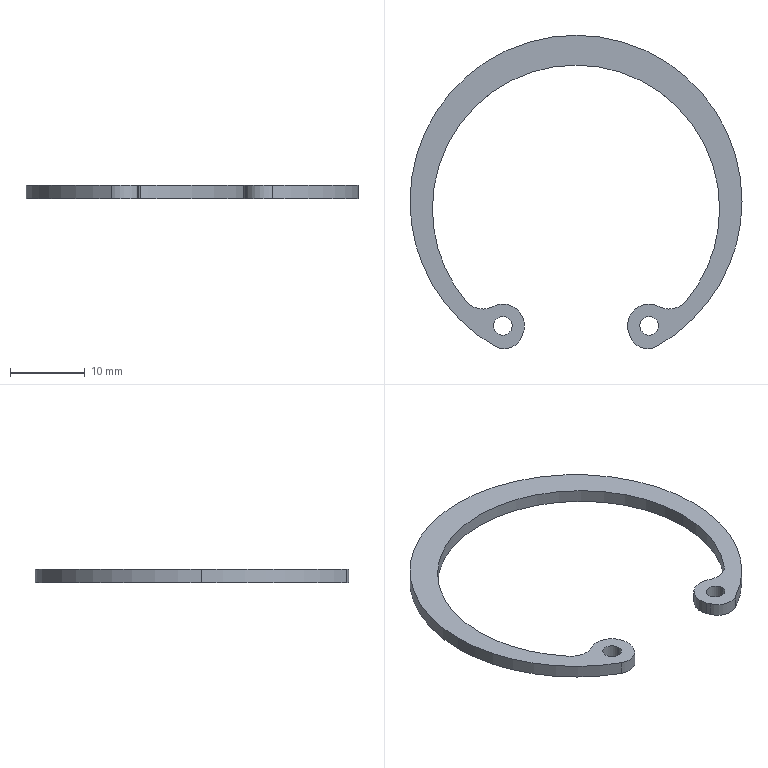Component | SolidWorks | Q1-A12-S21-Q1A.SLDASQ-1_Q1-BGSBB6004ZZ-40.sldasQ-1_Q1-RRING-C-INT-42-2 | 1 solid | 21 faces | box 44.5 x 42.01 x 1.75 mm | volume 670 mm3 | cylinder 17 | plane 4 | commonest cylinder face diameters 5.8 x5 2.5 x4 38.5 x3 44.5 x3 5 x2
build123d program:
from build123d import *

# Parameters (mm, degrees)
BOSS_EXTRUDE1_DEPTH      = 0.875
BOSS_EXTRUDE1_DEPTH_BACK = 0.875
SKETCH1_R                = 1.25


with BuildPart() as part:
    # Sketch1 → Boss-Extrude1 (new, two sides: drawn at the far end of the back side and taken through both)
    with BuildSketch(Plane(origin=(0, 0, 0), x_dir=(0, 0, -1), z_dir=(1, 0, 0)).offset(-BOSS_EXTRUDE1_DEPTH_BACK)):
        with BuildLine():
            Line((-7.278, -18.189), (-7.108, -17.762))
            ThreePointArc((-7.108, -17.762), (-7.857, -14.532), (-11.146, -14.116))
            ThreePointArc((-11.146, -14.116), (-13.05, -14.394), (-14.709, -13.419))
            ThreePointArc((-14.709, -13.419), (0, 18.25), (14.709, -13.419))
            ThreePointArc((14.709, -13.419), (13.05, -14.394), (11.146, -14.116))
            ThreePointArc((11.146, -14.116), (7.857, -14.532), (7.108, -17.762))
            Line((7.108, -17.762), (7.278, -18.189))
            ThreePointArc((7.278, -18.189), (8.763, -19.616), (10.815, -19.445))
            ThreePointArc((10.815, -19.445), (0, 22.25), (-10.815, -19.445))
            ThreePointArc((-10.815, -19.445), (-8.763, -19.616), (-7.278, -18.189))
        make_face()
        with Locations((9.8, -16.685)):
            Circle(SKETCH1_R, mode=Mode.SUBTRACT)
        with Locations((-9.8, -16.685)):
            Circle(SKETCH1_R, mode=Mode.SUBTRACT)
    extrude(amount=BOSS_EXTRUDE1_DEPTH + BOSS_EXTRUDE1_DEPTH_BACK)


solid = part.part

# Placed as in the assembly
solid = solid.moved(Location((0, 0, -170.425), (0, 90, 0)))
STEP:
#1=COLOUR_RGB('',0.7922,0.8196,0.9333);
#2=FILL_AREA_STYLE_COLOUR('',#1);
#3=FILL_AREA_STYLE('',(#2));
#4=SURFACE_STYLE_FILL_AREA(#3);
#5=SURFACE_SIDE_STYLE('',(#4));
#6=SURFACE_STYLE_USAGE(.BOTH.,#5);
#7=PRESENTATION_STYLE_ASSIGNMENT((#6));
#8=CARTESIAN_POINT('',(0.435,-0.6569,-6.744));
#9=VERTEX_POINT('',#8);
#10=CARTESIAN_POINT('',(0.3366,-0.6569,-6.744));
#11=VERTEX_POINT('',#10);
#12=CARTESIAN_POINT('',(0.3858,-0.6569,-6.744));
#13=DIRECTION('',(-0.,0.,-1.));
#14=DIRECTION('',(-1.,0.,0.));
#15=AXIS2_PLACEMENT_3D('',#12,#13,#14);
#16=CIRCLE('',#15,0.04921);
#17=EDGE_CURVE('',#9,#11,#16,.T.);
#18=ORIENTED_EDGE('',*,*,#17,.T.);
#19=CARTESIAN_POINT('',(0.3366,-0.6569,-6.675));
#20=VERTEX_POINT('',#19);
#21=CARTESIAN_POINT('',(0.3366,-0.6569,-6.744));
#22=DIRECTION('',(0.,-0.,1.));
#23=VECTOR('',#22,39.37);
#24=LINE('',#21,#23);
#25=EDGE_CURVE('',#11,#20,#24,.T.);
#26=ORIENTED_EDGE('',*,*,#25,.T.);
#27=CARTESIAN_POINT('',(0.435,-0.6569,-6.675));
#28=VERTEX_POINT('',#27);
#29=CARTESIAN_POINT('',(0.3858,-0.6569,-6.675));
#30=DIRECTION('',(-0.,0.,-1.));
#31=DIRECTION('',(-1.,0.,0.));
#32=AXIS2_PLACEMENT_3D('',#29,#30,#31);
#33=CIRCLE('',#32,0.04921);
#34=EDGE_CURVE('',#28,#20,#33,.T.);
#35=ORIENTED_EDGE('',*,*,#34,.F.);
#36=CARTESIAN_POINT('',(0.435,-0.6569,-6.744));
#37=DIRECTION('',(0.,-0.,1.));
#38=VECTOR('',#37,39.37);
#39=LINE('',#36,#38);
#40=EDGE_CURVE('',#9,#28,#39,.T.);
#41=ORIENTED_EDGE('',*,*,#40,.F.);
#42=EDGE_LOOP('',(#18,#26,#35,#41));
#43=FACE_OUTER_BOUND('',#42,.T.);
#44=CARTESIAN_POINT('',(0.3858,-0.6569,-6.744));
#45=DIRECTION('',(0.,-0.,1.));
#46=DIRECTION('',(1.,0.,0.));
#47=AXIS2_PLACEMENT_3D('',#44,#45,#46);
#48=CYLINDRICAL_SURFACE('',#47,0.04921);
#49=ADVANCED_FACE('',(#43),#48,.F.);
#50=CARTESIAN_POINT('',(-0.3366,-0.6569,-6.744));
#51=VERTEX_POINT('',#50);
#52=CARTESIAN_POINT('',(-0.435,-0.6569,-6.744));
#53=VERTEX_POINT('',#52);
#54=CARTESIAN_POINT('',(-0.3858,-0.6569,-6.744));
#55=DIRECTION('',(-0.,0.,-1.));
#56=DIRECTION('',(-1.,0.,0.));
#57=AXIS2_PLACEMENT_3D('',#54,#55,#56);
#58=CIRCLE('',#57,0.04921);
#59=EDGE_CURVE('',#51,#53,#58,.T.);
#60=ORIENTED_EDGE('',*,*,#59,.T.);
#61=CARTESIAN_POINT('',(-0.435,-0.6569,-6.675));
#62=VERTEX_POINT('',#61);
#63=CARTESIAN_POINT('',(-0.435,-0.6569,-6.744));
#64=DIRECTION('',(0.,-0.,1.));
#65=VECTOR('',#64,39.37);
#66=LINE('',#63,#65);
#67=EDGE_CURVE('',#53,#62,#66,.T.);
#68=ORIENTED_EDGE('',*,*,#67,.T.);
#69=CARTESIAN_POINT('',(-0.3366,-0.6569,-6.675));
#70=VERTEX_POINT('',#69);
#71=CARTESIAN_POINT('',(-0.3858,-0.6569,-6.675));
#72=DIRECTION('',(-0.,0.,-1.));
#73=DIRECTION('',(-1.,0.,0.));
#74=AXIS2_PLACEMENT_3D('',#71,#72,#73);
#75=CIRCLE('',#74,0.04921);
#76=EDGE_CURVE('',#70,#62,#75,.T.);
#77=ORIENTED_EDGE('',*,*,#76,.F.);
#78=CARTESIAN_POINT('',(-0.3366,-0.6569,-6.744));
#79=DIRECTION('',(0.,-0.,1.));
#80=VECTOR('',#79,39.37);
#81=LINE('',#78,#80);
#82=EDGE_CURVE('',#51,#70,#81,.T.);
#83=ORIENTED_EDGE('',*,*,#82,.F.);
#84=EDGE_LOOP('',(#60,#68,#77,#83));
#85=FACE_OUTER_BOUND('',#84,.T.);
#86=CARTESIAN_POINT('',(-0.3858,-0.6569,-6.744));
#87=DIRECTION('',(0.,-0.,1.));
#88=DIRECTION('',(1.,0.,0.));
#89=AXIS2_PLACEMENT_3D('',#86,#87,#88);
#90=CYLINDRICAL_SURFACE('',#89,0.04921);
#91=ADVANCED_FACE('',(#85),#90,.F.);
#92=CARTESIAN_POINT('',(-0.2717,-0.6569,-6.744));
#93=VERTEX_POINT('',#92);
#94=CARTESIAN_POINT('',(-0.2798,-0.6993,-6.744));
#95=VERTEX_POINT('',#94);
#96=CARTESIAN_POINT('',(-0.3858,-0.6569,-6.744));
#97=DIRECTION('',(-0.,0.,-1.));
#98=DIRECTION('',(-1.,0.,0.));
#99=AXIS2_PLACEMENT_3D('',#96,#97,#98);
#100=CIRCLE('',#99,0.1142);
#101=EDGE_CURVE('',#93,#95,#100,.T.);
#102=ORIENTED_EDGE('',*,*,#101,.F.);
#103=CARTESIAN_POINT('',(-0.2717,-0.6569,-6.675));
#104=VERTEX_POINT('',#103);
#105=CARTESIAN_POINT('',(-0.2717,-0.6569,-6.744));
#106=DIRECTION('',(0.,-0.,1.));
#107=VECTOR('',#106,39.37);
#108=LINE('',#105,#107);
#109=EDGE_CURVE('',#93,#104,#108,.T.);
#110=ORIENTED_EDGE('',*,*,#109,.T.);
#111=CARTESIAN_POINT('',(-0.2798,-0.6993,-6.675));
#112=VERTEX_POINT('',#111);
#113=CARTESIAN_POINT('',(-0.3858,-0.6569,-6.675));
#114=DIRECTION('',(-0.,0.,-1.));
#115=DIRECTION('',(-1.,0.,0.));
#116=AXIS2_PLACEMENT_3D('',#113,#114,#115);
#117=CIRCLE('',#116,0.1142);
#118=EDGE_CURVE('',#104,#112,#117,.T.);
#119=ORIENTED_EDGE('',*,*,#118,.T.);
#120=CARTESIAN_POINT('',(-0.2798,-0.6993,-6.744));
#121=DIRECTION('',(0.,-0.,1.));
#122=VECTOR('',#121,39.37);
#123=LINE('',#120,#122);
#124=EDGE_CURVE('',#95,#112,#123,.T.);
#125=ORIENTED_EDGE('',*,*,#124,.F.);
#126=EDGE_LOOP('',(#102,#110,#119,#125));
#127=FACE_OUTER_BOUND('',#126,.T.);
#128=CARTESIAN_POINT('',(-0.3858,-0.6569,-6.744));
#129=DIRECTION('',(0.,-0.,1.));
#130=DIRECTION('',(1.,0.,0.));
#131=AXIS2_PLACEMENT_3D('',#128,#129,#130);
#132=CYLINDRICAL_SURFACE('',#131,0.1142);
#133=ADVANCED_FACE('',(#127),#132,.T.);
#134=CARTESIAN_POINT('',(-0.7579,-0.03937,-6.744));
#135=VERTEX_POINT('',#134);
#136=CARTESIAN_POINT('',(-0.5791,-0.5283,-6.744));
#137=VERTEX_POINT('',#136);
#138=CARTESIAN_POINT('',(-0.,-0.03937,-6.744));
#139=DIRECTION('',(0.,-0.,1.));
#140=DIRECTION('',(1.,0.,0.));
#141=AXIS2_PLACEMENT_3D('',#138,#139,#140);
#142=CIRCLE('',#141,0.7579);
#143=EDGE_CURVE('',#135,#137,#142,.T.);
#144=ORIENTED_EDGE('',*,*,#143,.F.);
#145=CARTESIAN_POINT('',(-0.7579,-0.03937,-6.675));
#146=VERTEX_POINT('',#145);
#147=CARTESIAN_POINT('',(-0.7579,-0.03937,-6.744));
#148=DIRECTION('',(0.,-0.,1.));
#149=VECTOR('',#148,39.37);
#150=LINE('',#147,#149);
#151=EDGE_CURVE('',#135,#146,#150,.T.);
#152=ORIENTED_EDGE('',*,*,#151,.T.);
#153=CARTESIAN_POINT('',(-0.5791,-0.5283,-6.675));
#154=VERTEX_POINT('',#153);
#155=CARTESIAN_POINT('',(-0.,-0.03937,-6.675));
#156=DIRECTION('',(0.,-0.,1.));
#157=DIRECTION('',(1.,0.,0.));
#158=AXIS2_PLACEMENT_3D('',#155,#156,#157);
#159=CIRCLE('',#158,0.7579);
#160=EDGE_CURVE('',#146,#154,#159,.T.);
#161=ORIENTED_EDGE('',*,*,#160,.T.);
#162=CARTESIAN_POINT('',(-0.5791,-0.5283,-6.744));
#163=DIRECTION('',(0.,-0.,1.));
#164=VECTOR('',#163,39.37);
#165=LINE('',#162,#164);
#166=EDGE_CURVE('',#137,#154,#165,.T.);
#167=ORIENTED_EDGE('',*,*,#166,.F.);
#168=EDGE_LOOP('',(#144,#152,#161,#167));
#169=FACE_OUTER_BOUND('',#168,.T.);
#170=CARTESIAN_POINT('',(-0.,-0.03937,-6.744));
#171=DIRECTION('',(0.,-0.,1.));
#172=DIRECTION('',(1.,0.,0.));
#173=AXIS2_PLACEMENT_3D('',#170,#171,#172);
#174=CYLINDRICAL_SURFACE('',#173,0.7579);
#175=ADVANCED_FACE('',(#169),#174,.F.);
#176=ORIENTED_EDGE('',*,*,#151,.F.);
#177=CARTESIAN_POINT('',(0.7579,-0.03937,-6.744));
#178=VERTEX_POINT('',#177);
#179=CARTESIAN_POINT('',(-0.,-0.03937,-6.744));
#180=DIRECTION('',(0.,-0.,1.));
#181=DIRECTION('',(1.,0.,0.));
#182=AXIS2_PLACEMENT_3D('',#179,#180,#181);
#183=CIRCLE('',#182,0.7579);
#184=EDGE_CURVE('',#178,#135,#183,.T.);
#185=ORIENTED_EDGE('',*,*,#184,.F.);
#186=CARTESIAN_POINT('',(0.7579,-0.03937,-6.675));
#187=VERTEX_POINT('',#186);
#188=CARTESIAN_POINT('',(0.7579,-0.03937,-6.744));
#189=DIRECTION('',(0.,-0.,1.));
#190=VECTOR('',#189,39.37);
#191=LINE('',#188,#190);
#192=EDGE_CURVE('',#178,#187,#191,.T.);
#193=ORIENTED_EDGE('',*,*,#192,.T.);
#194=CARTESIAN_POINT('',(-0.,-0.03937,-6.675));
#195=DIRECTION('',(0.,-0.,1.));
#196=DIRECTION('',(1.,0.,0.));
#197=AXIS2_PLACEMENT_3D('',#194,#195,#196);
#198=CIRCLE('',#197,0.7579);
#199=EDGE_CURVE('',#187,#146,#198,.T.);
#200=ORIENTED_EDGE('',*,*,#199,.T.);
#201=EDGE_LOOP('',(#176,#185,#193,#200));
#202=FACE_OUTER_BOUND('',#201,.T.);
#203=CARTESIAN_POINT('',(-0.,-0.03937,-6.744));
#204=DIRECTION('',(0.,-0.,1.));
#205=DIRECTION('',(1.,0.,0.));
#206=AXIS2_PLACEMENT_3D('',#203,#204,#205);
#207=CYLINDRICAL_SURFACE('',#206,0.7579);
#208=ADVANCED_FACE('',(#202),#207,.F.);
#209=CARTESIAN_POINT('',(-0.876,0.,-6.744));
#210=VERTEX_POINT('',#209);
#211=CARTESIAN_POINT('',(0.876,0.,-6.744));
#212=VERTEX_POINT('',#211);
#213=CARTESIAN_POINT('',(-0.,0.,-6.744));
#214=DIRECTION('',(-0.,0.,-1.));
#215=DIRECTION('',(-1.,-0.,0.));
#216=AXIS2_PLACEMENT_3D('',#213,#214,#215);
#217=CIRCLE('',#216,0.876);
#218=EDGE_CURVE('',#210,#212,#217,.T.);
#219=ORIENTED_EDGE('',*,*,#218,.F.);
#220=CARTESIAN_POINT('',(-0.876,0.,-6.675));
#221=VERTEX_POINT('',#220);
#222=CARTESIAN_POINT('',(-0.876,0.,-6.744));
#223=DIRECTION('',(0.,-0.,1.));
#224=VECTOR('',#223,39.37);
#225=LINE('',#222,#224);
#226=EDGE_CURVE('',#210,#221,#225,.T.);
#227=ORIENTED_EDGE('',*,*,#226,.T.);
#228=CARTESIAN_POINT('',(0.876,0.,-6.675));
#229=VERTEX_POINT('',#228);
#230=CARTESIAN_POINT('',(-0.,0.,-6.675));
#231=DIRECTION('',(-0.,0.,-1.));
#232=DIRECTION('',(-1.,-0.,0.));
#233=AXIS2_PLACEMENT_3D('',#230,#231,#232);
#234=CIRCLE('',#233,0.876);
#235=EDGE_CURVE('',#221,#229,#234,.T.);
#236=ORIENTED_EDGE('',*,*,#235,.T.);
#237=CARTESIAN_POINT('',(0.876,0.,-6.744));
#238=DIRECTION('',(0.,-0.,1.));
#239=VECTOR('',#238,39.37);
#240=LINE('',#237,#239);
#241=EDGE_CURVE('',#212,#229,#240,.T.);
#242=ORIENTED_EDGE('',*,*,#241,.F.);
#243=EDGE_LOOP('',(#219,#227,#236,#242));
#244=FACE_OUTER_BOUND('',#243,.T.);
#245=CARTESIAN_POINT('',(-0.,0.,-6.744));
#246=DIRECTION('',(0.,-0.,1.));
#247=DIRECTION('',(1.,0.,0.));
#248=AXIS2_PLACEMENT_3D('',#245,#246,#247);
#249=CYLINDRICAL_SURFACE('',#248,0.876);
#250=ADVANCED_FACE('',(#244),#249,.T.);
#251=CARTESIAN_POINT('',(0.4258,-0.7656,-6.744));
#252=VERTEX_POINT('',#251);
#253=CARTESIAN_POINT('',(-0.,0.,-6.744));
#254=DIRECTION('',(-0.,0.,-1.));
#255=DIRECTION('',(-1.,-0.,0.));
#256=AXIS2_PLACEMENT_3D('',#253,#254,#255);
#257=CIRCLE('',#256,0.876);
#258=EDGE_CURVE('',#212,#252,#257,.T.);
#259=ORIENTED_EDGE('',*,*,#258,.F.);
#260=ORIENTED_EDGE('',*,*,#241,.T.);
#261=CARTESIAN_POINT('',(0.4258,-0.7656,-6.675));
#262=VERTEX_POINT('',#261);
#263=CARTESIAN_POINT('',(-0.,0.,-6.675));
#264=DIRECTION('',(-0.,0.,-1.));
#265=DIRECTION('',(-1.,-0.,0.));
#266=AXIS2_PLACEMENT_3D('',#263,#264,#265);
#267=CIRCLE('',#266,0.876);
#268=EDGE_CURVE('',#229,#262,#267,.T.);
#269=ORIENTED_EDGE('',*,*,#268,.T.);
#270=CARTESIAN_POINT('',(0.4258,-0.7656,-6.744));
#271=DIRECTION('',(0.,-0.,1.));
#272=VECTOR('',#271,39.37);
#273=LINE('',#270,#272);
#274=EDGE_CURVE('',#252,#262,#273,.T.);
#275=ORIENTED_EDGE('',*,*,#274,.F.);
#276=EDGE_LOOP('',(#259,#260,#269,#275));
#277=FACE_OUTER_BOUND('',#276,.T.);
#278=CARTESIAN_POINT('',(-0.,0.,-6.744));
#279=DIRECTION('',(0.,-0.,1.));
#280=DIRECTION('',(1.,0.,0.));
#281=AXIS2_PLACEMENT_3D('',#278,#279,#280);
#282=CYLINDRICAL_SURFACE('',#281,0.876);
#283=ADVANCED_FACE('',(#277),#282,.T.);
#284=ORIENTED_EDGE('',*,*,#59,.F.);
#285=CARTESIAN_POINT('',(-0.3858,-0.6569,-6.744));
#286=DIRECTION('',(-0.,0.,-1.));
#287=DIRECTION('',(-1.,0.,0.));
#288=AXIS2_PLACEMENT_3D('',#285,#286,#287);
#289=CIRCLE('',#288,0.04921);
#290=EDGE_CURVE('',#53,#51,#289,.T.);
#291=ORIENTED_EDGE('',*,*,#290,.F.);
#292=EDGE_LOOP('',(#284,#291));
#293=FACE_BOUND('',#292,.T.);
#294=CARTESIAN_POINT('',(-0.2865,-0.7161,-6.744));
#295=VERTEX_POINT('',#294);
#296=CARTESIAN_POINT('',(-0.4258,-0.7656,-6.744));
#297=VERTEX_POINT('',#296);
#298=CARTESIAN_POINT('',(-0.3779,-0.6795,-6.744));
#299=DIRECTION('',(-0.,0.,-1.));
#300=DIRECTION('',(-1.,0.,0.));
#301=AXIS2_PLACEMENT_3D('',#298,#299,#300);
#302=CIRCLE('',#301,0.09843);
#303=EDGE_CURVE('',#295,#297,#302,.T.);
#304=ORIENTED_EDGE('',*,*,#303,.T.);
#305=CARTESIAN_POINT('',(-0.,0.,-6.744));
#306=DIRECTION('',(-0.,0.,-1.));
#307=DIRECTION('',(-1.,-0.,0.));
#308=AXIS2_PLACEMENT_3D('',#305,#306,#307);
#309=CIRCLE('',#308,0.876);
#310=EDGE_CURVE('',#297,#210,#309,.T.);
#311=ORIENTED_EDGE('',*,*,#310,.T.);
#312=ORIENTED_EDGE('',*,*,#218,.T.);
#313=ORIENTED_EDGE('',*,*,#258,.T.);
#314=CARTESIAN_POINT('',(0.2865,-0.7161,-6.744));
#315=VERTEX_POINT('',#314);
#316=CARTESIAN_POINT('',(0.3779,-0.6795,-6.744));
#317=DIRECTION('',(-0.,0.,-1.));
#318=DIRECTION('',(-1.,0.,0.));
#319=AXIS2_PLACEMENT_3D('',#316,#317,#318);
#320=CIRCLE('',#319,0.09843);
#321=EDGE_CURVE('',#252,#315,#320,.T.);
#322=ORIENTED_EDGE('',*,*,#321,.T.);
#323=CARTESIAN_POINT('',(0.2798,-0.6993,-6.744));
#324=VERTEX_POINT('',#323);
#325=CARTESIAN_POINT('',(0.2865,-0.7161,-6.744));
#326=DIRECTION('',(-0.3715,0.9284,0.));
#327=VECTOR('',#326,39.37);
#328=LINE('',#325,#327);
#329=EDGE_CURVE('',#315,#324,#328,.T.);
#330=ORIENTED_EDGE('',*,*,#329,.T.);
#331=CARTESIAN_POINT('',(0.4388,-0.5558,-6.744));
#332=VERTEX_POINT('',#331);
#333=CARTESIAN_POINT('',(0.3858,-0.6569,-6.744));
#334=DIRECTION('',(-0.,0.,-1.));
#335=DIRECTION('',(-1.,0.,0.));
#336=AXIS2_PLACEMENT_3D('',#333,#334,#335);
#337=CIRCLE('',#336,0.1142);
#338=EDGE_CURVE('',#324,#332,#337,.T.);
#339=ORIENTED_EDGE('',*,*,#338,.T.);
#340=CARTESIAN_POINT('',(0.5791,-0.5283,-6.744));
#341=VERTEX_POINT('',#340);
#342=CARTESIAN_POINT('',(0.4918,-0.4546,-6.744));
#343=DIRECTION('',(0.,-0.,1.));
#344=DIRECTION('',(1.,0.,0.));
#345=AXIS2_PLACEMENT_3D('',#342,#343,#344);
#346=CIRCLE('',#345,0.1142);
#347=EDGE_CURVE('',#332,#341,#346,.T.);
#348=ORIENTED_EDGE('',*,*,#347,.T.);
#349=CARTESIAN_POINT('',(-0.,-0.03937,-6.744));
#350=DIRECTION('',(0.,-0.,1.));
#351=DIRECTION('',(1.,0.,0.));
#352=AXIS2_PLACEMENT_3D('',#349,#350,#351);
#353=CIRCLE('',#352,0.7579);
#354=EDGE_CURVE('',#341,#178,#353,.T.);
#355=ORIENTED_EDGE('',*,*,#354,.T.);
#356=ORIENTED_EDGE('',*,*,#184,.T.);
#357=ORIENTED_EDGE('',*,*,#143,.T.);
#358=CARTESIAN_POINT('',(-0.4388,-0.5558,-6.744));
#359=VERTEX_POINT('',#358);
#360=CARTESIAN_POINT('',(-0.4918,-0.4546,-6.744));
#361=DIRECTION('',(0.,-0.,1.));
#362=DIRECTION('',(1.,0.,0.));
#363=AXIS2_PLACEMENT_3D('',#360,#361,#362);
#364=CIRCLE('',#363,0.1142);
#365=EDGE_CURVE('',#137,#359,#364,.T.);
#366=ORIENTED_EDGE('',*,*,#365,.T.);
#367=CARTESIAN_POINT('',(-0.3858,-0.6569,-6.744));
#368=DIRECTION('',(-0.,0.,-1.));
#369=DIRECTION('',(-1.,0.,0.));
#370=AXIS2_PLACEMENT_3D('',#367,#368,#369);
#371=CIRCLE('',#370,0.1142);
#372=EDGE_CURVE('',#359,#93,#371,.T.);
#373=ORIENTED_EDGE('',*,*,#372,.T.);
#374=ORIENTED_EDGE('',*,*,#101,.T.);
#375=CARTESIAN_POINT('',(-0.2798,-0.6993,-6.744));
#376=DIRECTION('',(-0.3715,-0.9284,-0.));
#377=VECTOR('',#376,39.37);
#378=LINE('',#375,#377);
#379=EDGE_CURVE('',#95,#295,#378,.T.);
#380=ORIENTED_EDGE('',*,*,#379,.T.);
#381=EDGE_LOOP('',(#304,#311,#312,#313,#322,#330,#339,#348,#355,#356,#357,#366,#373,#374,#380));
#382=FACE_OUTER_BOUND('',#381,.T.);
#383=ORIENTED_EDGE('',*,*,#17,.F.);
#384=CARTESIAN_POINT('',(0.3858,-0.6569,-6.744));
#385=DIRECTION('',(-0.,0.,-1.));
#386=DIRECTION('',(-1.,0.,0.));
#387=AXIS2_PLACEMENT_3D('',#384,#385,#386);
#388=CIRCLE('',#387,0.04921);
#389=EDGE_CURVE('',#11,#9,#388,.T.);
#390=ORIENTED_EDGE('',*,*,#389,.F.);
#391=EDGE_LOOP('',(#383,#390));
#392=FACE_BOUND('',#391,.T.);
#393=CARTESIAN_POINT('',(-0.3779,-0.6795,-6.744));
#394=DIRECTION('',(0.,0.,-1.));
#395=DIRECTION('',(-1.,-0.,-0.));
#396=AXIS2_PLACEMENT_3D('',#393,#394,#395);
#397=PLANE('',#396);
#398=ADVANCED_FACE('',(#293,#382,#392),#397,.T.);
#399=CARTESIAN_POINT('',(-0.2865,-0.7161,-6.675));
#400=VERTEX_POINT('',#399);
#401=CARTESIAN_POINT('',(-0.2865,-0.7161,-6.744));
#402=DIRECTION('',(0.,-0.,1.));
#403=VECTOR('',#402,39.37);
#404=LINE('',#401,#403);
#405=EDGE_CURVE('',#295,#400,#404,.T.);
#406=ORIENTED_EDGE('',*,*,#405,.T.);
#407=CARTESIAN_POINT('',(-0.4258,-0.7656,-6.675));
#408=VERTEX_POINT('',#407);
#409=CARTESIAN_POINT('',(-0.3779,-0.6795,-6.675));
#410=DIRECTION('',(-0.,0.,-1.));
#411=DIRECTION('',(-1.,0.,0.));
#412=AXIS2_PLACEMENT_3D('',#409,#410,#411);
#413=CIRCLE('',#412,0.09843);
#414=EDGE_CURVE('',#400,#408,#413,.T.);
#415=ORIENTED_EDGE('',*,*,#414,.T.);
#416=CARTESIAN_POINT('',(-0.4258,-0.7656,-6.744));
#417=DIRECTION('',(0.,-0.,1.));
#418=VECTOR('',#417,39.37);
#419=LINE('',#416,#418);
#420=EDGE_CURVE('',#297,#408,#419,.T.);
#421=ORIENTED_EDGE('',*,*,#420,.F.);
#422=ORIENTED_EDGE('',*,*,#303,.F.);
#423=EDGE_LOOP('',(#406,#415,#421,#422));
#424=FACE_OUTER_BOUND('',#423,.T.);
#425=CARTESIAN_POINT('',(-0.3779,-0.6795,-6.744));
#426=DIRECTION('',(0.,-0.,1.));
#427=DIRECTION('',(1.,0.,0.));
#428=AXIS2_PLACEMENT_3D('',#425,#426,#427);
#429=CYLINDRICAL_SURFACE('',#428,0.09843);
#430=ADVANCED_FACE('',(#424),#429,.T.);
#431=ORIENTED_EDGE('',*,*,#226,.F.);
#432=ORIENTED_EDGE('',*,*,#310,.F.);
#433=ORIENTED_EDGE('',*,*,#420,.T.);
#434=CARTESIAN_POINT('',(-0.,0.,-6.675));
#435=DIRECTION('',(-0.,0.,-1.));
#436=DIRECTION('',(-1.,-0.,0.));
#437=AXIS2_PLACEMENT_3D('',#434,#435,#436);
#438=CIRCLE('',#437,0.876);
#439=EDGE_CURVE('',#408,#221,#438,.T.);
#440=ORIENTED_EDGE('',*,*,#439,.T.);
#441=EDGE_LOOP('',(#431,#432,#433,#440));
#442=FACE_OUTER_BOUND('',#441,.T.);
#443=CARTESIAN_POINT('',(-0.,0.,-6.744));
#444=DIRECTION('',(0.,-0.,1.));
#445=DIRECTION('',(1.,0.,0.));
#446=AXIS2_PLACEMENT_3D('',#443,#444,#445);
#447=CYLINDRICAL_SURFACE('',#446,0.876);
#448=ADVANCED_FACE('',(#442),#447,.T.);
#449=ORIENTED_EDGE('',*,*,#274,.T.);
#450=CARTESIAN_POINT('',(0.2865,-0.7161,-6.675));
#451=VERTEX_POINT('',#450);
#452=CARTESIAN_POINT('',(0.3779,-0.6795,-6.675));
#453=DIRECTION('',(-0.,0.,-1.));
#454=DIRECTION('',(-1.,0.,0.));
#455=AXIS2_PLACEMENT_3D('',#452,#453,#454);
#456=CIRCLE('',#455,0.09843);
#457=EDGE_CURVE('',#262,#451,#456,.T.);
#458=ORIENTED_EDGE('',*,*,#457,.T.);
#459=CARTESIAN_POINT('',(0.2865,-0.7161,-6.744));
#460=DIRECTION('',(0.,-0.,1.));
#461=VECTOR('',#460,39.37);
#462=LINE('',#459,#461);
#463=EDGE_CURVE('',#315,#451,#462,.T.);
#464=ORIENTED_EDGE('',*,*,#463,.F.);
#465=ORIENTED_EDGE('',*,*,#321,.F.);
#466=EDGE_LOOP('',(#449,#458,#464,#465));
#467=FACE_OUTER_BOUND('',#466,.T.);
#468=CARTESIAN_POINT('',(0.3779,-0.6795,-6.744));
#469=DIRECTION('',(0.,-0.,1.));
#470=DIRECTION('',(1.,0.,0.));
#471=AXIS2_PLACEMENT_3D('',#468,#469,#470);
#472=CYLINDRICAL_SURFACE('',#471,0.09843);
#473=ADVANCED_FACE('',(#467),#472,.T.);
#474=ORIENTED_EDGE('',*,*,#463,.T.);
#475=CARTESIAN_POINT('',(0.2798,-0.6993,-6.675));
#476=VERTEX_POINT('',#475);
#477=CARTESIAN_POINT('',(0.2865,-0.7161,-6.675));
#478=DIRECTION('',(-0.3715,0.9284,0.));
#479=VECTOR('',#478,39.37);
#480=LINE('',#477,#479);
#481=EDGE_CURVE('',#451,#476,#480,.T.);
#482=ORIENTED_EDGE('',*,*,#481,.T.);
#483=CARTESIAN_POINT('',(0.2798,-0.6993,-6.744));
#484=DIRECTION('',(0.,-0.,1.));
#485=VECTOR('',#484,39.37);
#486=LINE('',#483,#485);
#487=EDGE_CURVE('',#324,#476,#486,.T.);
#488=ORIENTED_EDGE('',*,*,#487,.F.);
#489=ORIENTED_EDGE('',*,*,#329,.F.);
#490=EDGE_LOOP('',(#474,#482,#488,#489));
#491=FACE_OUTER_BOUND('',#490,.T.);
#492=CARTESIAN_POINT('',(0.2865,-0.7161,-6.744));
#493=DIRECTION('',(0.9284,0.3715,0.));
#494=DIRECTION('',(0.3715,-0.9284,-0.));
#495=AXIS2_PLACEMENT_3D('',#492,#493,#494);
#496=PLANE('',#495);
#497=ADVANCED_FACE('',(#491),#496,.F.);
#498=ORIENTED_EDGE('',*,*,#487,.T.);
#499=CARTESIAN_POINT('',(0.4388,-0.5558,-6.675));
#500=VERTEX_POINT('',#499);
#501=CARTESIAN_POINT('',(0.3858,-0.6569,-6.675));
#502=DIRECTION('',(-0.,0.,-1.));
#503=DIRECTION('',(-1.,0.,0.));
#504=AXIS2_PLACEMENT_3D('',#501,#502,#503);
#505=CIRCLE('',#504,0.1142);
#506=EDGE_CURVE('',#476,#500,#505,.T.);
#507=ORIENTED_EDGE('',*,*,#506,.T.);
#508=CARTESIAN_POINT('',(0.4388,-0.5558,-6.744));
#509=DIRECTION('',(0.,-0.,1.));
#510=VECTOR('',#509,39.37);
#511=LINE('',#508,#510);
#512=EDGE_CURVE('',#332,#500,#511,.T.);
#513=ORIENTED_EDGE('',*,*,#512,.F.);
#514=ORIENTED_EDGE('',*,*,#338,.F.);
#515=EDGE_LOOP('',(#498,#507,#513,#514));
#516=FACE_OUTER_BOUND('',#515,.T.);
#517=CARTESIAN_POINT('',(0.3858,-0.6569,-6.744));
#518=DIRECTION('',(0.,-0.,1.));
#519=DIRECTION('',(1.,0.,0.));
#520=AXIS2_PLACEMENT_3D('',#517,#518,#519);
#521=CYLINDRICAL_SURFACE('',#520,0.1142);
#522=ADVANCED_FACE('',(#516),#521,.T.);
#523=ORIENTED_EDGE('',*,*,#512,.T.);
#524=CARTESIAN_POINT('',(0.5791,-0.5283,-6.675));
#525=VERTEX_POINT('',#524);
#526=CARTESIAN_POINT('',(0.4918,-0.4546,-6.675));
#527=DIRECTION('',(0.,-0.,1.));
#528=DIRECTION('',(1.,0.,0.));
#529=AXIS2_PLACEMENT_3D('',#526,#527,#528);
#530=CIRCLE('',#529,0.1142);
#531=EDGE_CURVE('',#500,#525,#530,.T.);
#532=ORIENTED_EDGE('',*,*,#531,.T.);
#533=CARTESIAN_POINT('',(0.5791,-0.5283,-6.744));
#534=DIRECTION('',(0.,-0.,1.));
#535=VECTOR('',#534,39.37);
#536=LINE('',#533,#535);
#537=EDGE_CURVE('',#341,#525,#536,.T.);
#538=ORIENTED_EDGE('',*,*,#537,.F.);
#539=ORIENTED_EDGE('',*,*,#347,.F.);
#540=EDGE_LOOP('',(#523,#532,#538,#539));
#541=FACE_OUTER_BOUND('',#540,.T.);
#542=CARTESIAN_POINT('',(0.4918,-0.4546,-6.744));
#543=DIRECTION('',(0.,-0.,1.));
#544=DIRECTION('',(1.,0.,0.));
#545=AXIS2_PLACEMENT_3D('',#542,#543,#544);
#546=CYLINDRICAL_SURFACE('',#545,0.1142);
#547=ADVANCED_FACE('',(#541),#546,.F.);
#548=ORIENTED_EDGE('',*,*,#192,.F.);
#549=ORIENTED_EDGE('',*,*,#354,.F.);
#550=ORIENTED_EDGE('',*,*,#537,.T.);
#551=CARTESIAN_POINT('',(-0.,-0.03937,-6.675));
#552=DIRECTION('',(0.,-0.,1.));
#553=DIRECTION('',(1.,0.,0.));
#554=AXIS2_PLACEMENT_3D('',#551,#552,#553);
#555=CIRCLE('',#554,0.7579);
#556=EDGE_CURVE('',#525,#187,#555,.T.);
#557=ORIENTED_EDGE('',*,*,#556,.T.);
#558=EDGE_LOOP('',(#548,#549,#550,#557));
#559=FACE_OUTER_BOUND('',#558,.T.);
#560=CARTESIAN_POINT('',(-0.,-0.03937,-6.744));
#561=DIRECTION('',(0.,-0.,1.));
#562=DIRECTION('',(1.,0.,0.));
#563=AXIS2_PLACEMENT_3D('',#560,#561,#562);
#564=CYLINDRICAL_SURFACE('',#563,0.7579);
#565=ADVANCED_FACE('',(#559),#564,.F.);
#566=ORIENTED_EDGE('',*,*,#166,.T.);
#567=CARTESIAN_POINT('',(-0.4388,-0.5558,-6.675));
#568=VERTEX_POINT('',#567);
#569=CARTESIAN_POINT('',(-0.4918,-0.4546,-6.675));
#570=DIRECTION('',(0.,-0.,1.));
#571=DIRECTION('',(1.,0.,0.));
#572=AXIS2_PLACEMENT_3D('',#569,#570,#571);
#573=CIRCLE('',#572,0.1142);
#574=EDGE_CURVE('',#154,#568,#573,.T.);
#575=ORIENTED_EDGE('',*,*,#574,.T.);
#576=CARTESIAN_POINT('',(-0.4388,-0.5558,-6.744));
#577=DIRECTION('',(0.,-0.,1.));
#578=VECTOR('',#577,39.37);
#579=LINE('',#576,#578);
#580=EDGE_CURVE('',#359,#568,#579,.T.);
#581=ORIENTED_EDGE('',*,*,#580,.F.);
#582=ORIENTED_EDGE('',*,*,#365,.F.);
#583=EDGE_LOOP('',(#566,#575,#581,#582));
#584=FACE_OUTER_BOUND('',#583,.T.);
#585=CARTESIAN_POINT('',(-0.4918,-0.4546,-6.744));
#586=DIRECTION('',(0.,-0.,1.));
#587=DIRECTION('',(1.,0.,0.));
#588=AXIS2_PLACEMENT_3D('',#585,#586,#587);
#589=CYLINDRICAL_SURFACE('',#588,0.1142);
#590=ADVANCED_FACE('',(#584),#589,.F.);
#591=ORIENTED_EDGE('',*,*,#109,.F.);
#592=ORIENTED_EDGE('',*,*,#372,.F.);
#593=ORIENTED_EDGE('',*,*,#580,.T.);
#594=CARTESIAN_POINT('',(-0.3858,-0.6569,-6.675));
#595=DIRECTION('',(-0.,0.,-1.));
#596=DIRECTION('',(-1.,0.,0.));
#597=AXIS2_PLACEMENT_3D('',#594,#595,#596);
#598=CIRCLE('',#597,0.1142);
#599=EDGE_CURVE('',#568,#104,#598,.T.);
#600=ORIENTED_EDGE('',*,*,#599,.T.);
#601=EDGE_LOOP('',(#591,#592,#593,#600));
#602=FACE_OUTER_BOUND('',#601,.T.);
#603=CARTESIAN_POINT('',(-0.3858,-0.6569,-6.744));
#604=DIRECTION('',(0.,-0.,1.));
#605=DIRECTION('',(1.,0.,0.));
#606=AXIS2_PLACEMENT_3D('',#603,#604,#605);
#607=CYLINDRICAL_SURFACE('',#606,0.1142);
#608=ADVANCED_FACE('',(#602),#607,.T.);
#609=ORIENTED_EDGE('',*,*,#124,.T.);
#610=CARTESIAN_POINT('',(-0.2798,-0.6993,-6.675));
#611=DIRECTION('',(-0.3715,-0.9284,-0.));
#612=VECTOR('',#611,39.37);
#613=LINE('',#610,#612);
#614=EDGE_CURVE('',#112,#400,#613,.T.);
#615=ORIENTED_EDGE('',*,*,#614,.T.);
#616=ORIENTED_EDGE('',*,*,#405,.F.);
#617=ORIENTED_EDGE('',*,*,#379,.F.);
#618=EDGE_LOOP('',(#609,#615,#616,#617));
#619=FACE_OUTER_BOUND('',#618,.T.);
#620=CARTESIAN_POINT('',(-0.2798,-0.6993,-6.744));
#621=DIRECTION('',(-0.9284,0.3715,0.));
#622=DIRECTION('',(0.3715,0.9284,0.));
#623=AXIS2_PLACEMENT_3D('',#620,#621,#622);
#624=PLANE('',#623);
#625=ADVANCED_FACE('',(#619),#624,.F.);
#626=ORIENTED_EDGE('',*,*,#67,.F.);
#627=ORIENTED_EDGE('',*,*,#290,.T.);
#628=ORIENTED_EDGE('',*,*,#82,.T.);
#629=CARTESIAN_POINT('',(-0.3858,-0.6569,-6.675));
#630=DIRECTION('',(-0.,0.,-1.));
#631=DIRECTION('',(-1.,0.,0.));
#632=AXIS2_PLACEMENT_3D('',#629,#630,#631);
#633=CIRCLE('',#632,0.04921);
#634=EDGE_CURVE('',#62,#70,#633,.T.);
#635=ORIENTED_EDGE('',*,*,#634,.F.);
#636=EDGE_LOOP('',(#626,#627,#628,#635));
#637=FACE_OUTER_BOUND('',#636,.T.);
#638=CARTESIAN_POINT('',(-0.3858,-0.6569,-6.744));
#639=DIRECTION('',(0.,-0.,1.));
#640=DIRECTION('',(1.,0.,0.));
#641=AXIS2_PLACEMENT_3D('',#638,#639,#640);
#642=CYLINDRICAL_SURFACE('',#641,0.04921);
#643=ADVANCED_FACE('',(#637),#642,.F.);
#644=ORIENTED_EDGE('',*,*,#25,.F.);
#645=ORIENTED_EDGE('',*,*,#389,.T.);
#646=ORIENTED_EDGE('',*,*,#40,.T.);
#647=CARTESIAN_POINT('',(0.3858,-0.6569,-6.675));
#648=DIRECTION('',(-0.,0.,-1.));
#649=DIRECTION('',(-1.,0.,0.));
#650=AXIS2_PLACEMENT_3D('',#647,#648,#649);
#651=CIRCLE('',#650,0.04921);
#652=EDGE_CURVE('',#20,#28,#651,.T.);
#653=ORIENTED_EDGE('',*,*,#652,.F.);
#654=EDGE_LOOP('',(#644,#645,#646,#653));
#655=FACE_OUTER_BOUND('',#654,.T.);
#656=CARTESIAN_POINT('',(0.3858,-0.6569,-6.744));
#657=DIRECTION('',(0.,-0.,1.));
#658=DIRECTION('',(1.,0.,0.));
#659=AXIS2_PLACEMENT_3D('',#656,#657,#658);
#660=CYLINDRICAL_SURFACE('',#659,0.04921);
#661=ADVANCED_FACE('',(#655),#660,.F.);
#662=ORIENTED_EDGE('',*,*,#34,.T.);
#663=ORIENTED_EDGE('',*,*,#652,.T.);
#664=EDGE_LOOP('',(#662,#663));
#665=FACE_BOUND('',#664,.T.);
#666=ORIENTED_EDGE('',*,*,#76,.T.);
#667=ORIENTED_EDGE('',*,*,#634,.T.);
#668=EDGE_LOOP('',(#666,#667));
#669=FACE_BOUND('',#668,.T.);
#670=ORIENTED_EDGE('',*,*,#414,.F.);
#671=ORIENTED_EDGE('',*,*,#614,.F.);
#672=ORIENTED_EDGE('',*,*,#118,.F.);
#673=ORIENTED_EDGE('',*,*,#599,.F.);
#674=ORIENTED_EDGE('',*,*,#574,.F.);
#675=ORIENTED_EDGE('',*,*,#160,.F.);
#676=ORIENTED_EDGE('',*,*,#199,.F.);
#677=ORIENTED_EDGE('',*,*,#556,.F.);
#678=ORIENTED_EDGE('',*,*,#531,.F.);
#679=ORIENTED_EDGE('',*,*,#506,.F.);
#680=ORIENTED_EDGE('',*,*,#481,.F.);
#681=ORIENTED_EDGE('',*,*,#457,.F.);
#682=ORIENTED_EDGE('',*,*,#268,.F.);
#683=ORIENTED_EDGE('',*,*,#235,.F.);
#684=ORIENTED_EDGE('',*,*,#439,.F.);
#685=EDGE_LOOP('',(#670,#671,#672,#673,#674,#675,#676,#677,#678,#679,#680,#681,#682,#683,#684));
#686=FACE_OUTER_BOUND('',#685,.T.);
#687=CARTESIAN_POINT('',(-0.3779,-0.6795,-6.675));
#688=DIRECTION('',(0.,0.,-1.));
#689=DIRECTION('',(-1.,-0.,-0.));
#690=AXIS2_PLACEMENT_3D('',#687,#688,#689);
#691=PLANE('',#690);
#692=ADVANCED_FACE('',(#665,#669,#686),#691,.F.);
#693=CLOSED_SHELL('',(#49,#91,#133,#175,#208,#250,#283,#398,#430,#448,#473,#497,#522,#547,#565,#590,#608,#625,#643,#661,#692));
#694=MANIFOLD_SOLID_BREP('',#693);
#695=STYLED_ITEM('',(#7),#694);
#696=(LENGTH_UNIT()NAMED_UNIT(*)SI_UNIT($,.METRE.));
#697=LENGTH_MEASURE_WITH_UNIT(LENGTH_MEASURE(0.0254),#696);
#698=DIMENSIONAL_EXPONENTS(1.,0.,0.,0.,0.,0.,0.);
#699=(CONVERSION_BASED_UNIT('',#697)LENGTH_UNIT()NAMED_UNIT(#698));
#700=UNCERTAINTY_MEASURE_WITH_UNIT(LENGTH_MEASURE(0.00001),#699,'','');
#701=(NAMED_UNIT(*)PLANE_ANGLE_UNIT()SI_UNIT($,.RADIAN.));
#702=(NAMED_UNIT(*)SI_UNIT($,.STERADIAN.)SOLID_ANGLE_UNIT());
#703=(GEOMETRIC_REPRESENTATION_CONTEXT(3)GLOBAL_UNCERTAINTY_ASSIGNED_CONTEXT((#700))GLOBAL_UNIT_ASSIGNED_CONTEXT((#699,#701,#702))REPRESENTATION_CONTEXT('',''));
#704=MECHANICAL_DESIGN_GEOMETRIC_PRESENTATION_REPRESENTATION('',(#695),#703);
#705=PRESENTATION_LAYER_ASSIGNMENT('','',(#695));
#706=CARTESIAN_POINT('',(0.,0.,0.));
#707=DIRECTION('',(0.,0.,1.));
#708=DIRECTION('',(1.,0.,0.));
#709=AXIS2_PLACEMENT_3D('',#706,#707,#708);
#710=(LENGTH_UNIT()NAMED_UNIT(*)SI_UNIT($,.METRE.));
#711=LENGTH_MEASURE_WITH_UNIT(LENGTH_MEASURE(0.0254),#710);
#712=DIMENSIONAL_EXPONENTS(1.,0.,0.,0.,0.,0.,0.);
#713=(CONVERSION_BASED_UNIT('',#711)LENGTH_UNIT()NAMED_UNIT(#712));
#714=UNCERTAINTY_MEASURE_WITH_UNIT(LENGTH_MEASURE(0.00001),#713,'','');
#715=(NAMED_UNIT(*)PLANE_ANGLE_UNIT()SI_UNIT($,.RADIAN.));
#716=(NAMED_UNIT(*)SI_UNIT($,.STERADIAN.)SOLID_ANGLE_UNIT());
#717=(GEOMETRIC_REPRESENTATION_CONTEXT(3)GLOBAL_UNCERTAINTY_ASSIGNED_CONTEXT((#714))GLOBAL_UNIT_ASSIGNED_CONTEXT((#713,#715,#716))REPRESENTATION_CONTEXT('',''));
#718=ADVANCED_BREP_SHAPE_REPRESENTATION('',(#694,#709),#717);